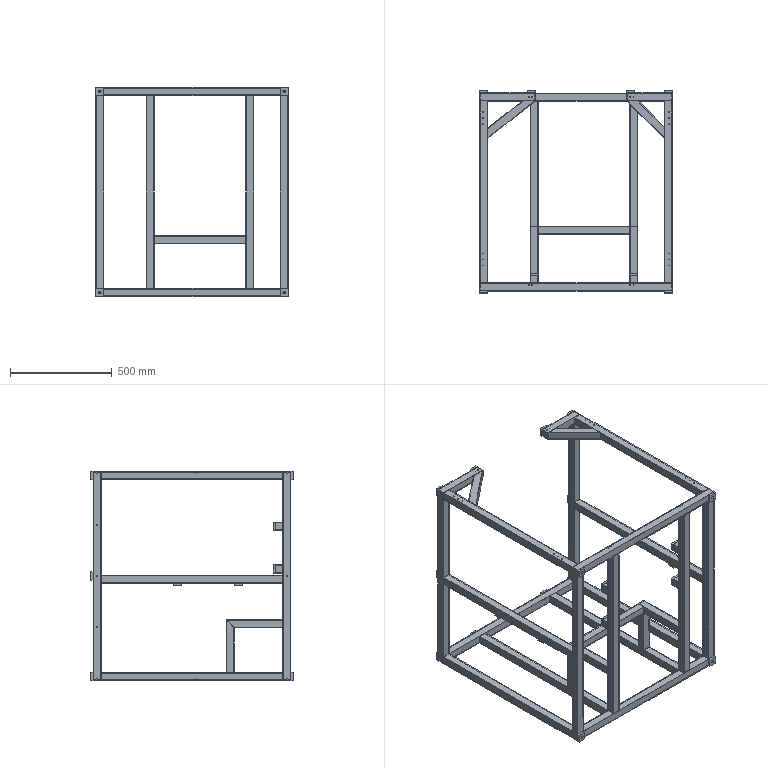Component | SolidWorks | SYM0671-81-101-1_SYM0671-81-101-2 | 54 solids | 640 faces | volume 8406900 mm3 | plane 444 | cylinder 196 | commonest cylinder face diameters 4.2 x68 8.5 x44 14 x28 3.3 x24 2.5 x16 6.8 x16 | material AISI 304